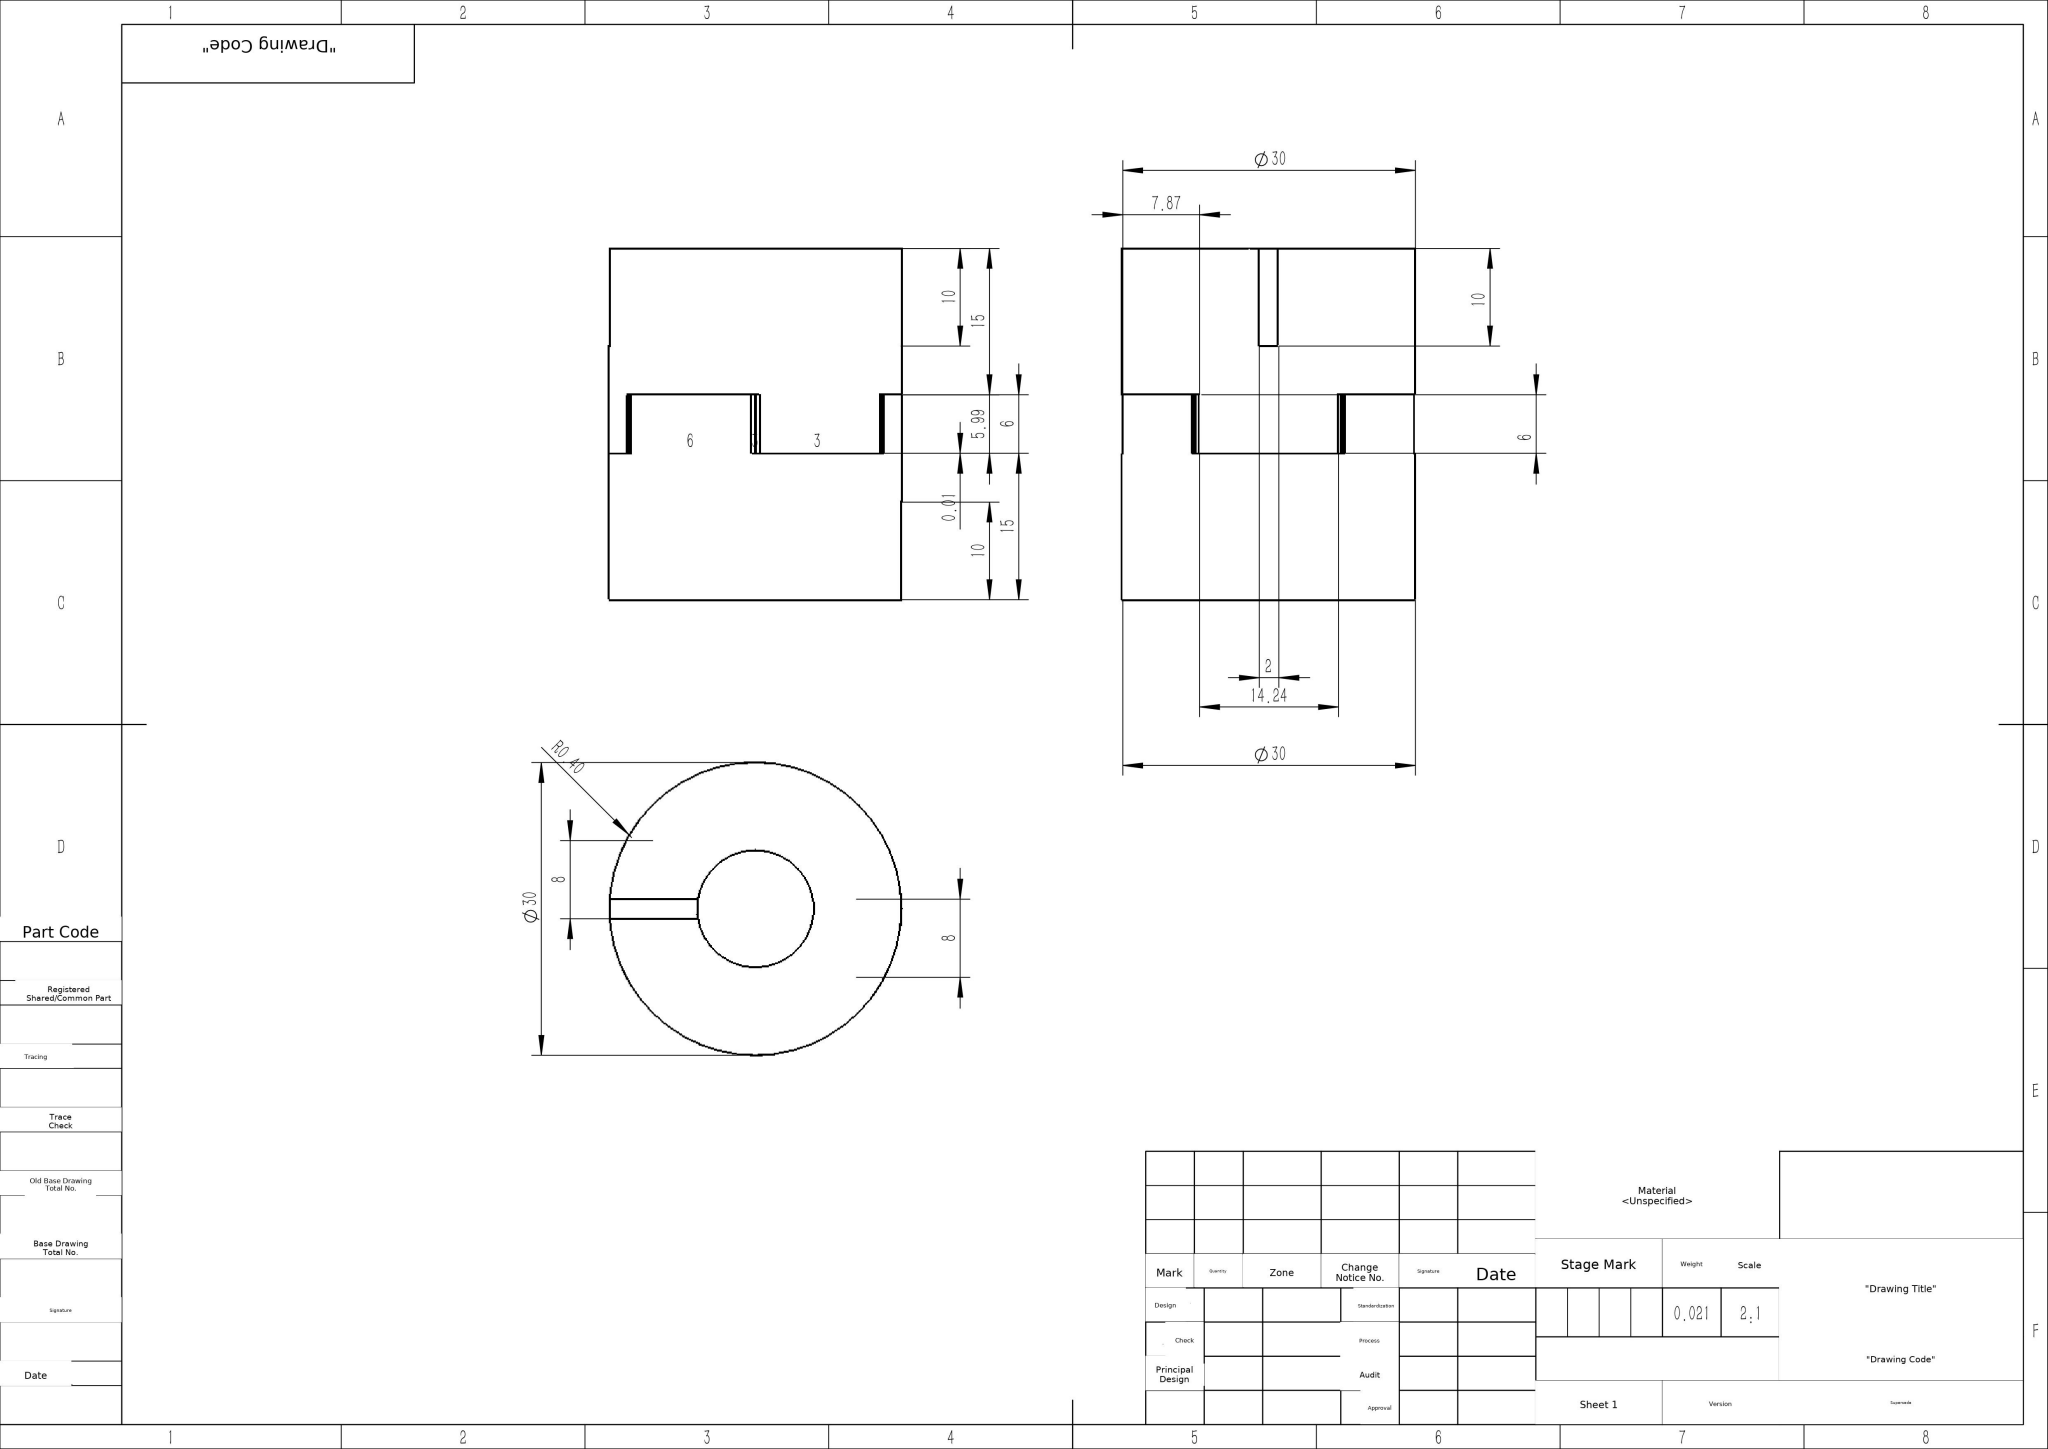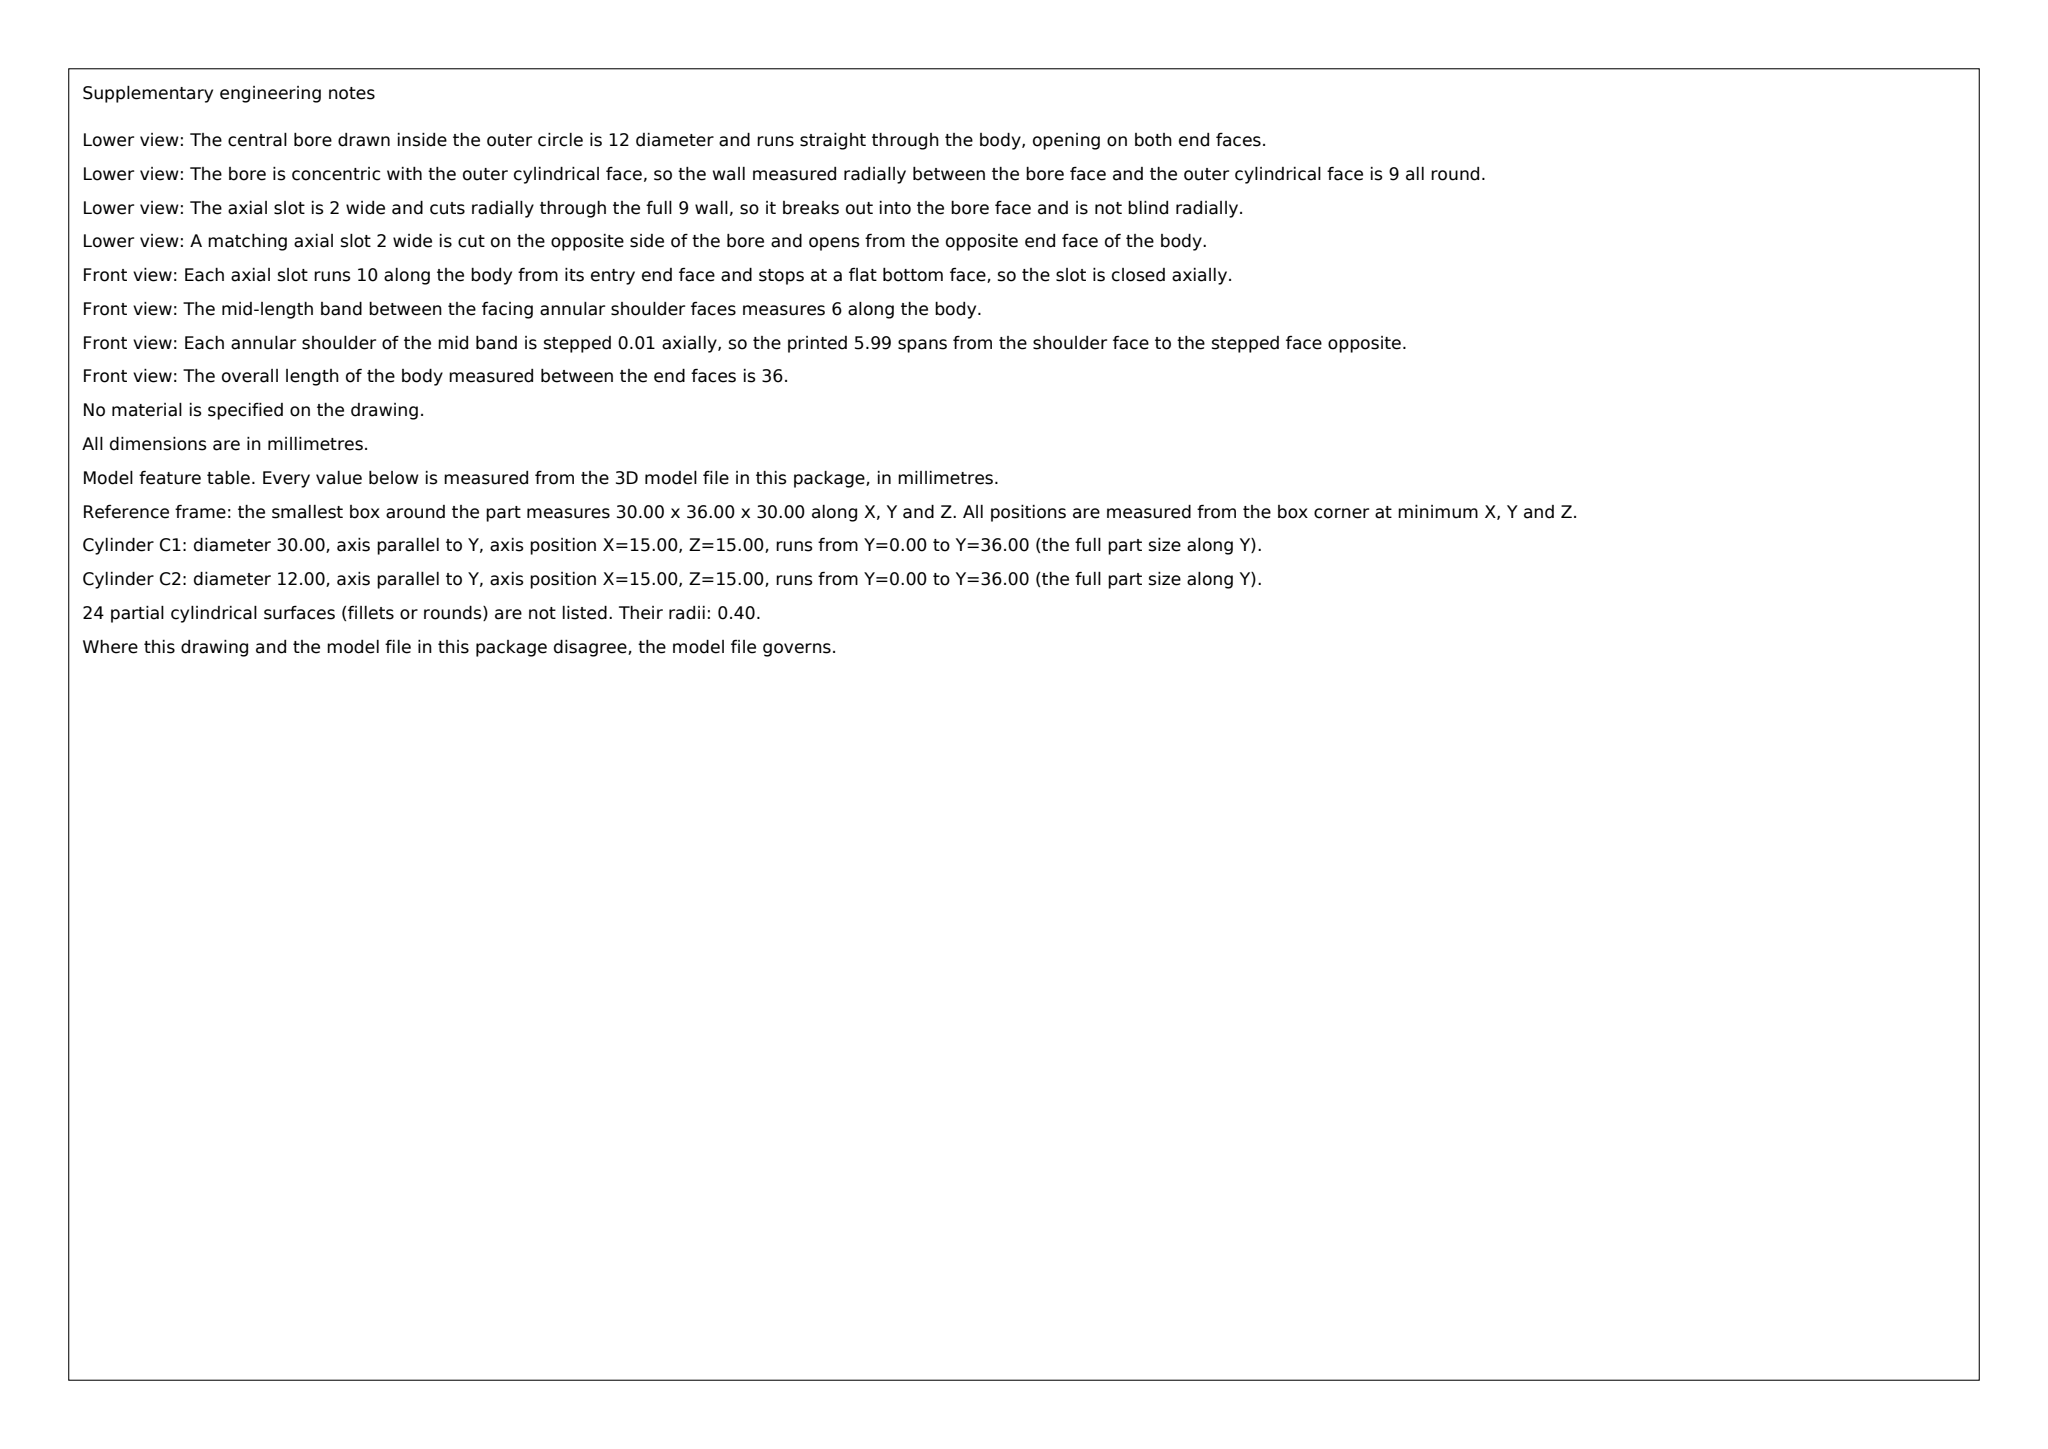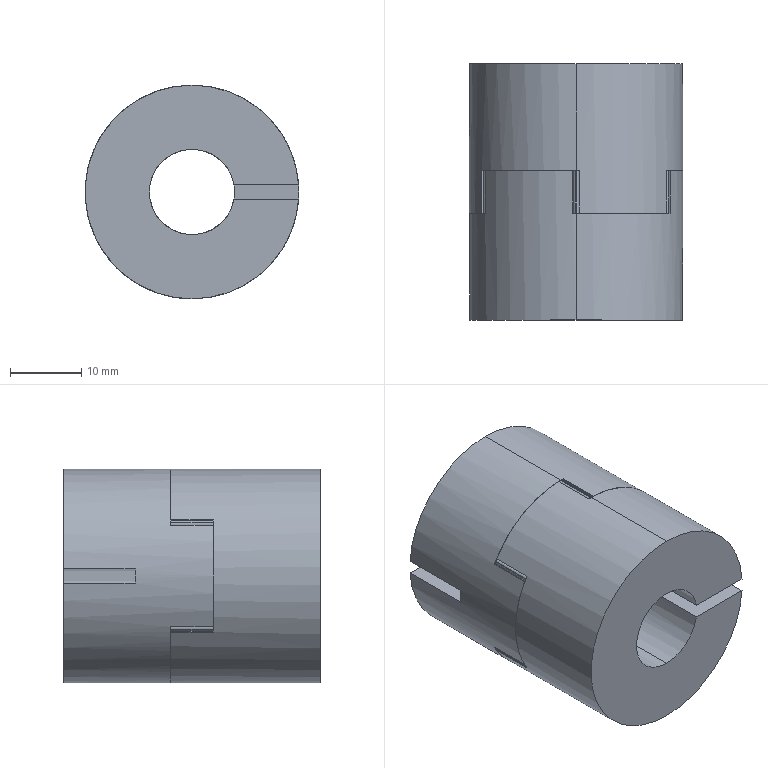Part | SolidWorks | mm | 1 solid | 108 faces | box 30 x 36 x 30 mm | volume 21004 mm3 | plane 74 | cylinder 34 | commonest cylinder face diameters 0.8 x28 30 x4 12 x2
Drawing notes:
Ø12 THRU BORE, COAXIAL W/ Ø30 OD | from the solid: cylinder dia 12, axis y, pos (15,15), length 36 = full bbox height
SLOT WIDTH 0.86 | from the solid: axis planes x=14.57 and x=15.43 -> 15.43-14.57=0.86
6 RADIAL SLOTS 0.86 WD EQ SP 60° ON Ø30 BAND | from the solid: 0.8 end-fillet pairs at 6 angular positions 60° apart about (15,15)
SLOT PATTERN: 1ST SLOT CL 30° CCW FROM HORIZ CL | from the solid: slot end centers at angles 30,90,150,210,270,330 from +x axis thru (15,15)
SLOT RADIAL EXTENT R5.98 (INTO BORE) TO R14.99 AT OD | from the solid: R0.4 fillet centers at r=6.38 and r=14.59 from axis -> 6.38-0.4, 14.59+0.4
SLOT CORNERS R0.40 TYP (4 PER SLOT) | from the solid: 24 cylinders dia 0.8, axis y, length 6
SLOTTED BAND 6 WD, 15 FROM EA END FACE, 36 OAL | from the solid: y planes 0, 15, 21, 36; slot cylinders length 6 spanning y=15 to 21